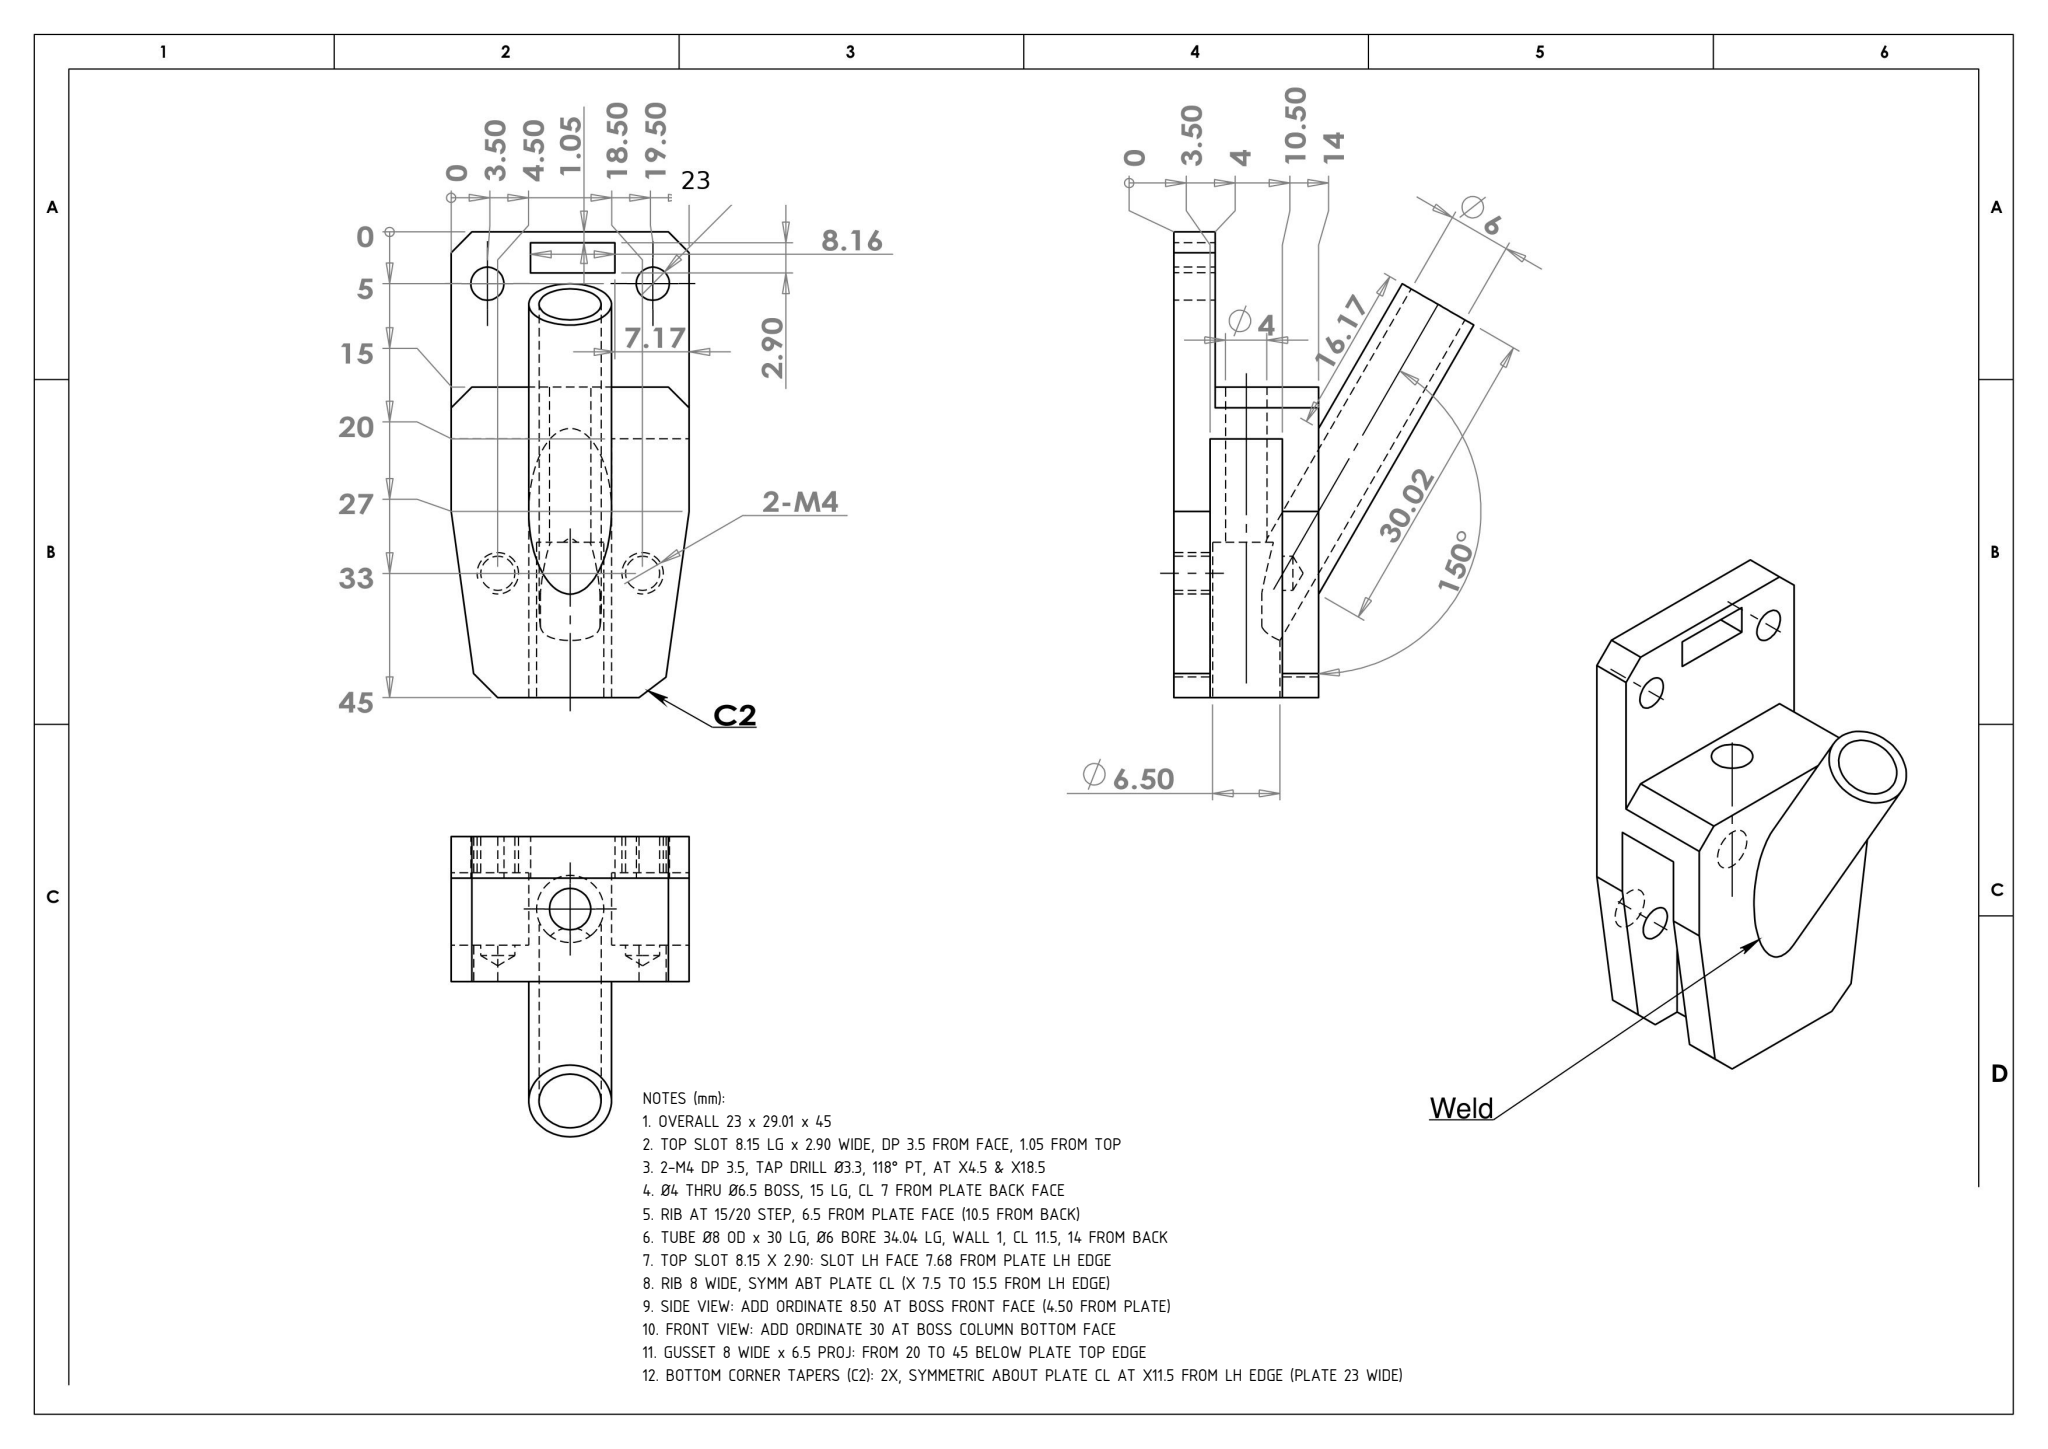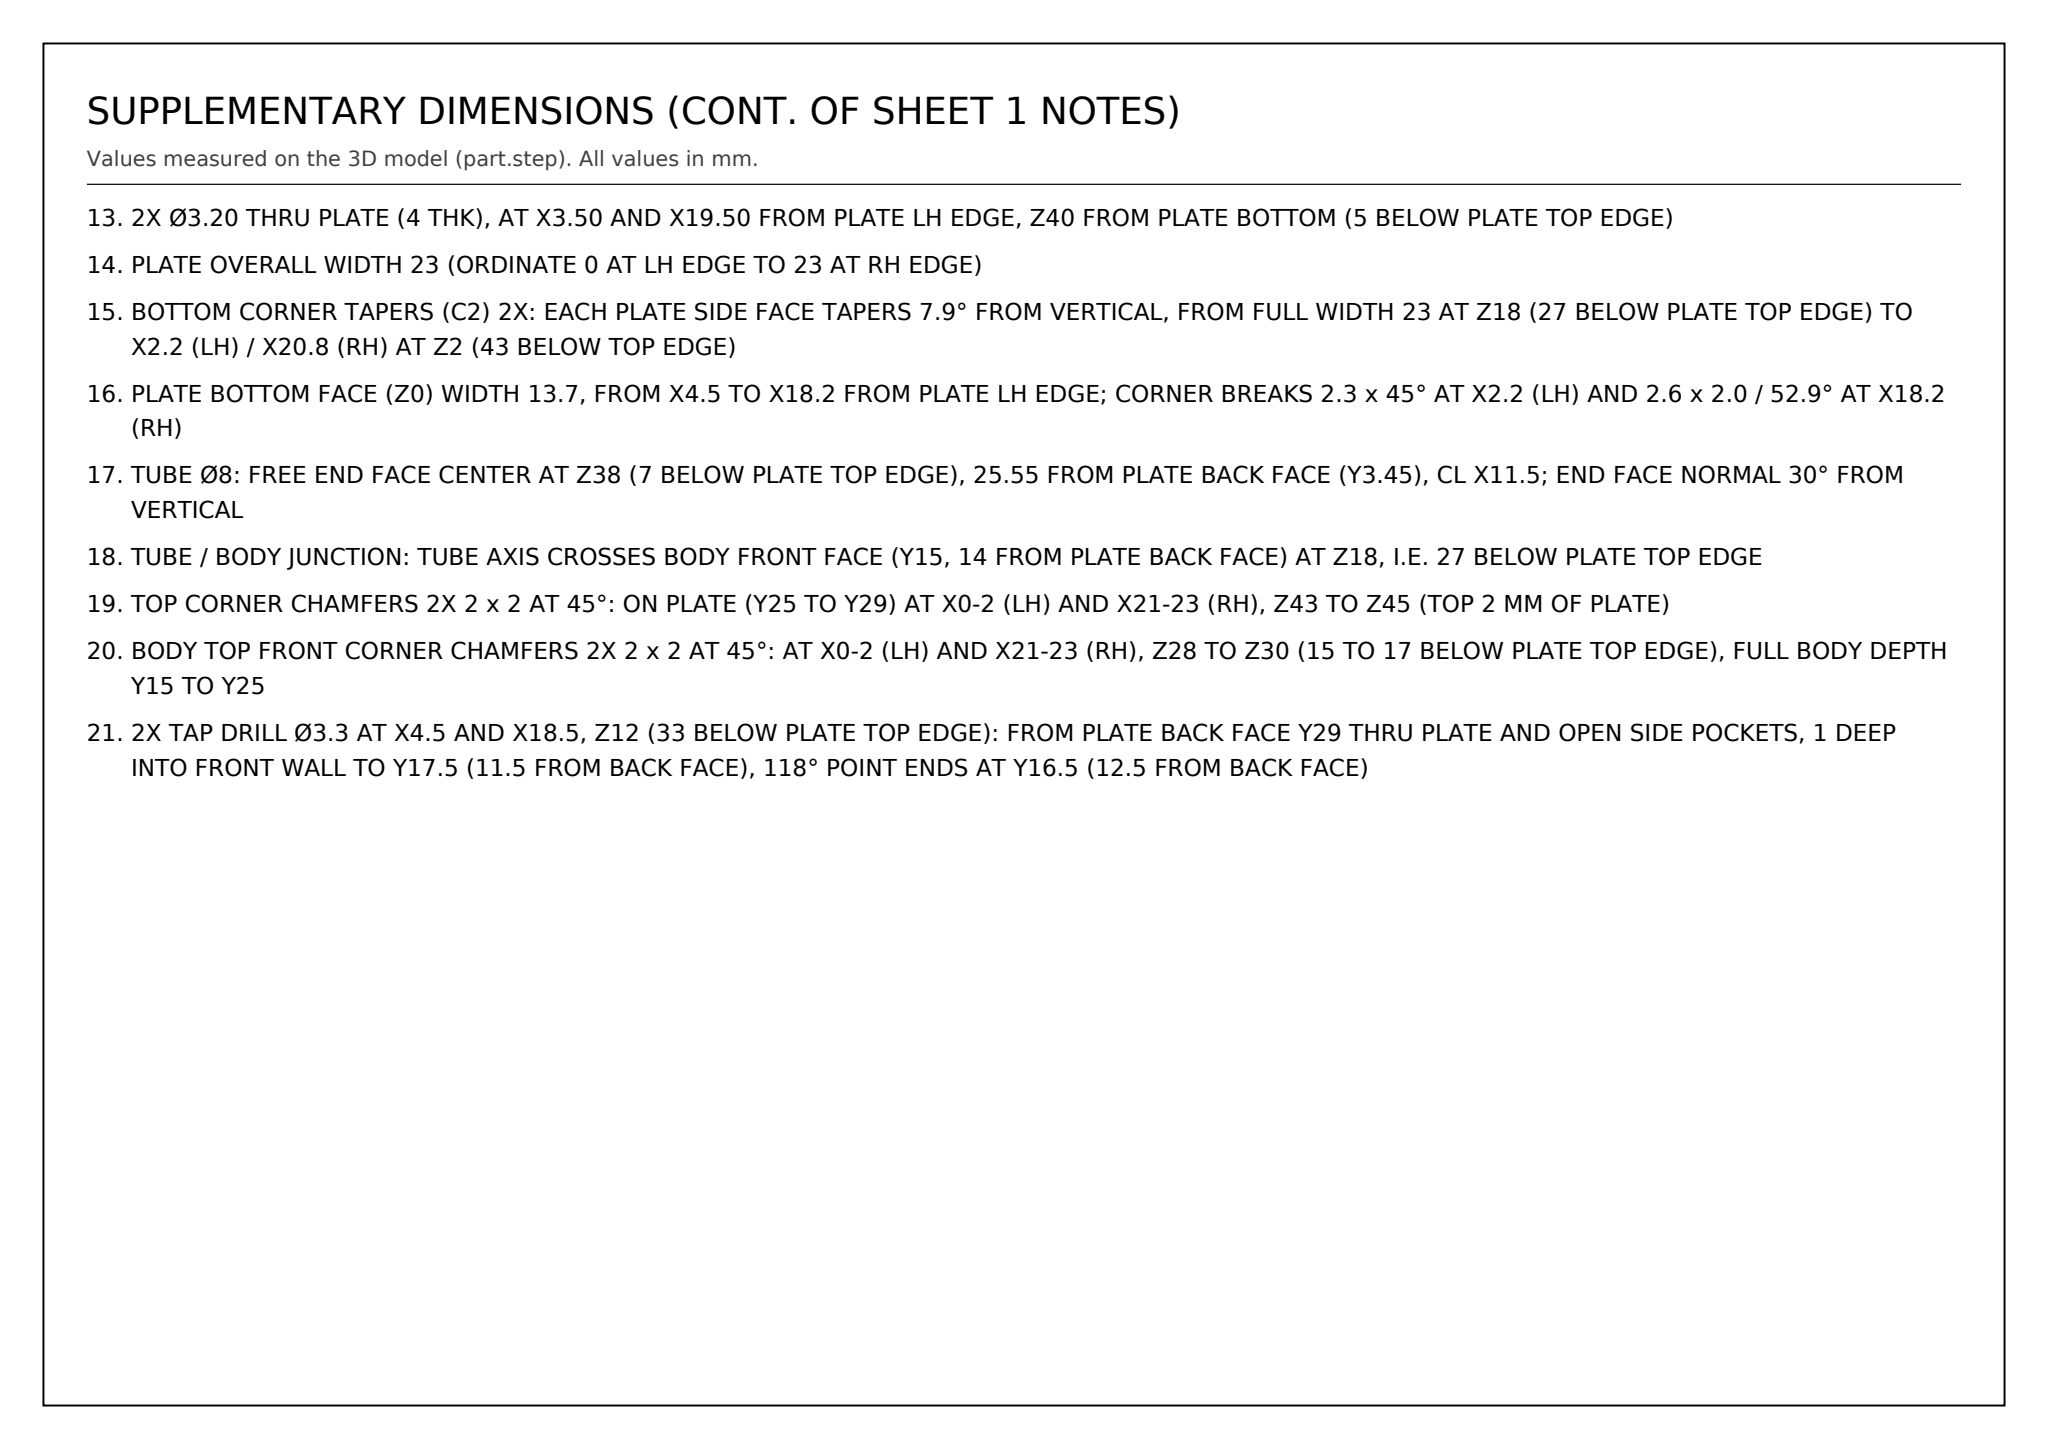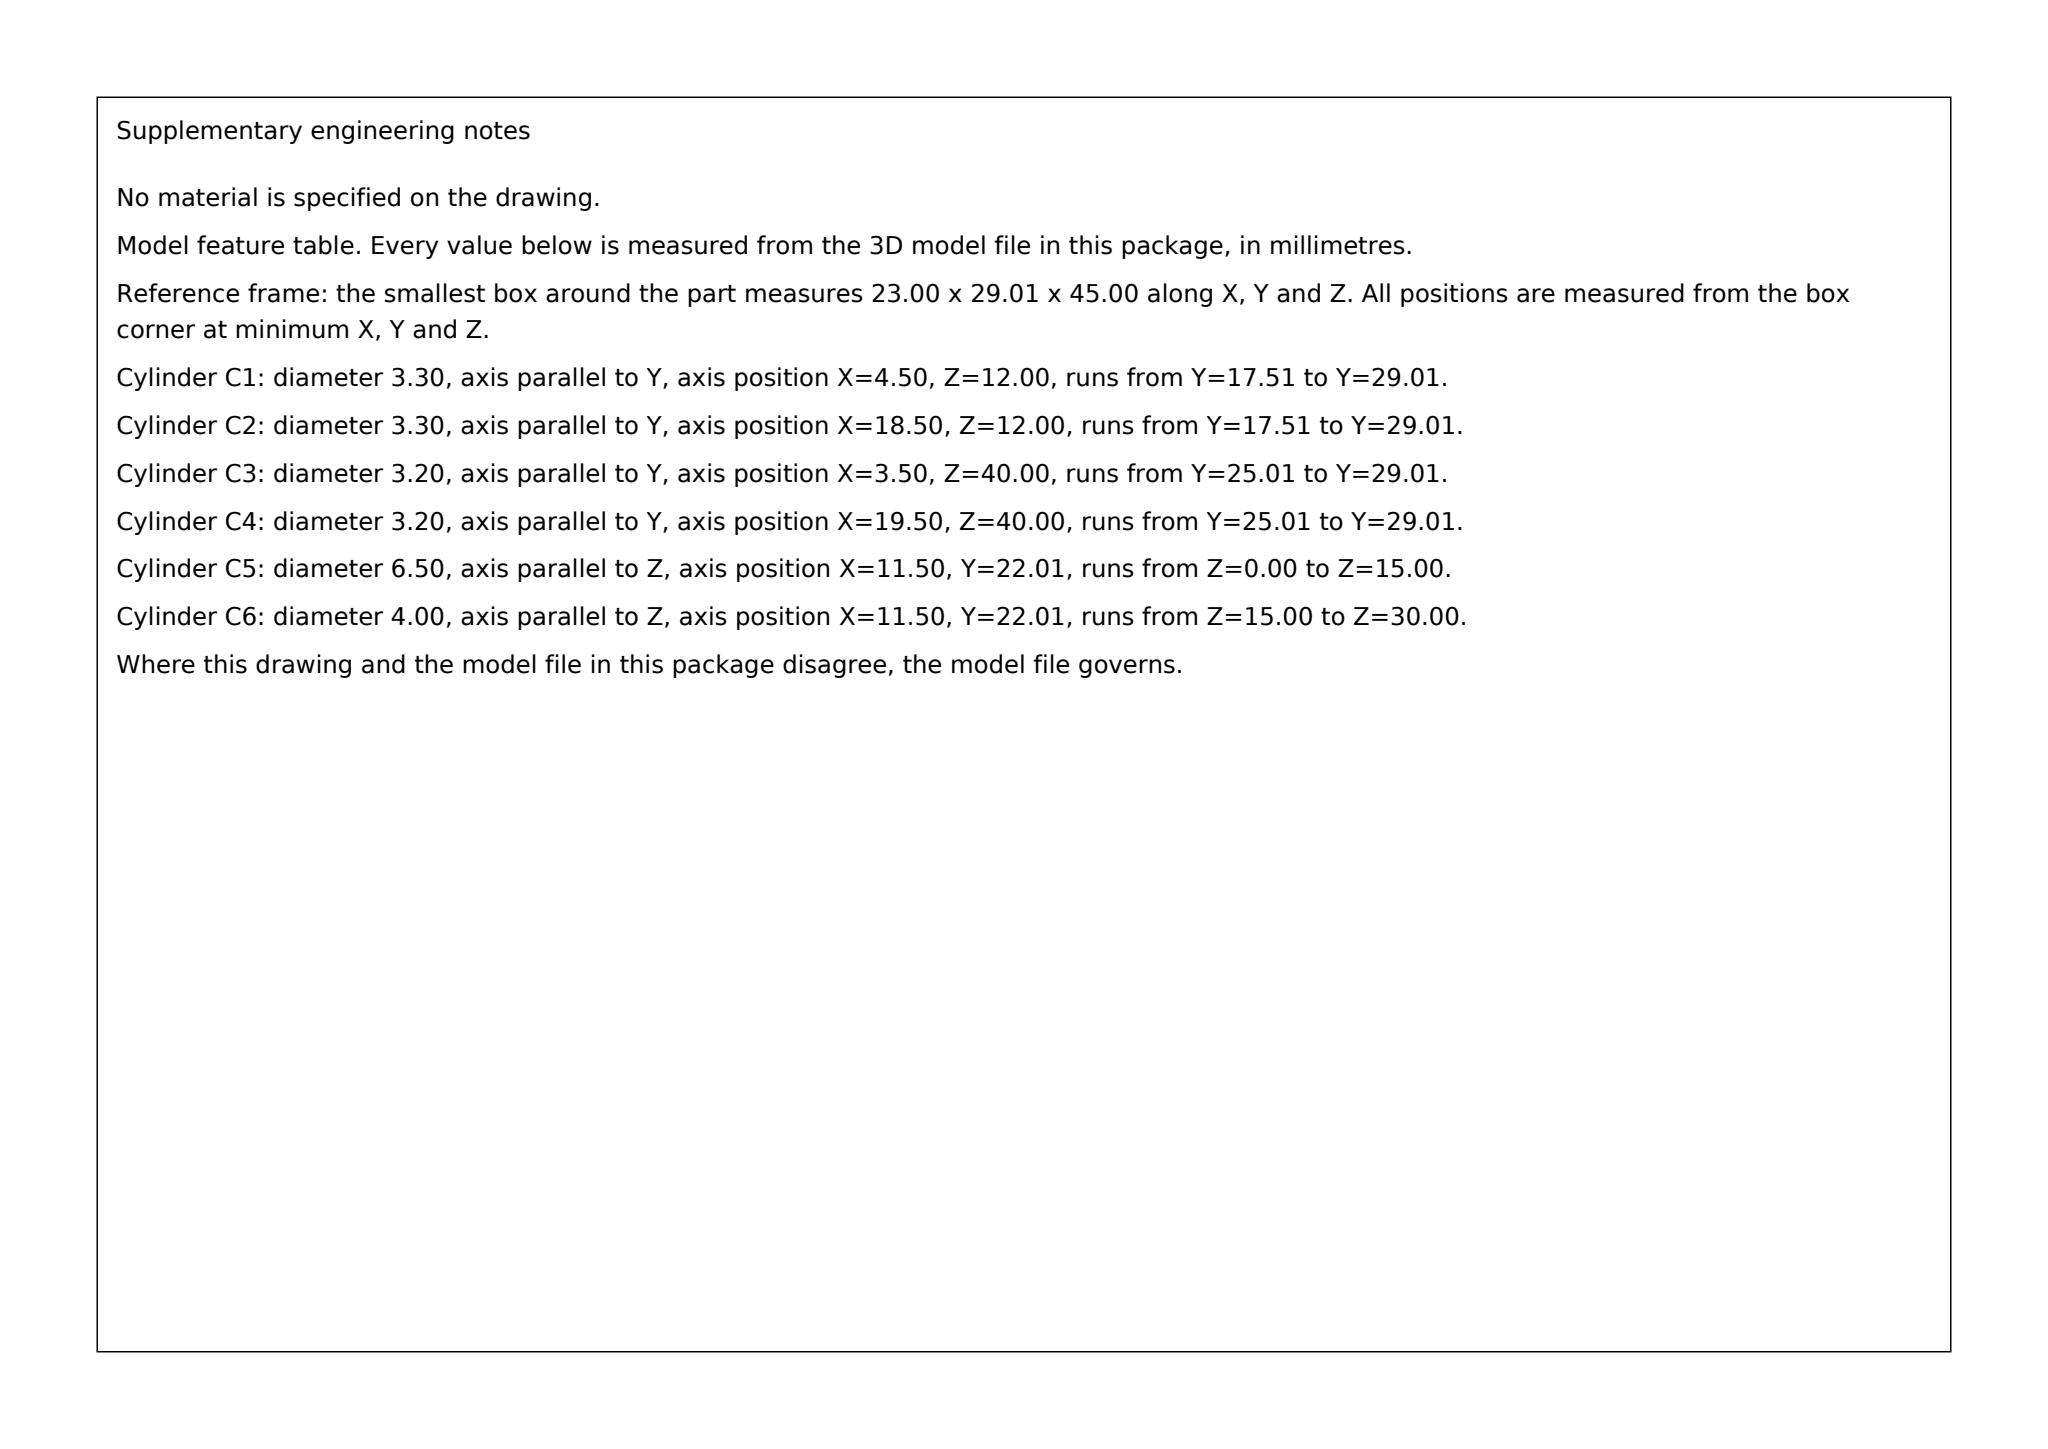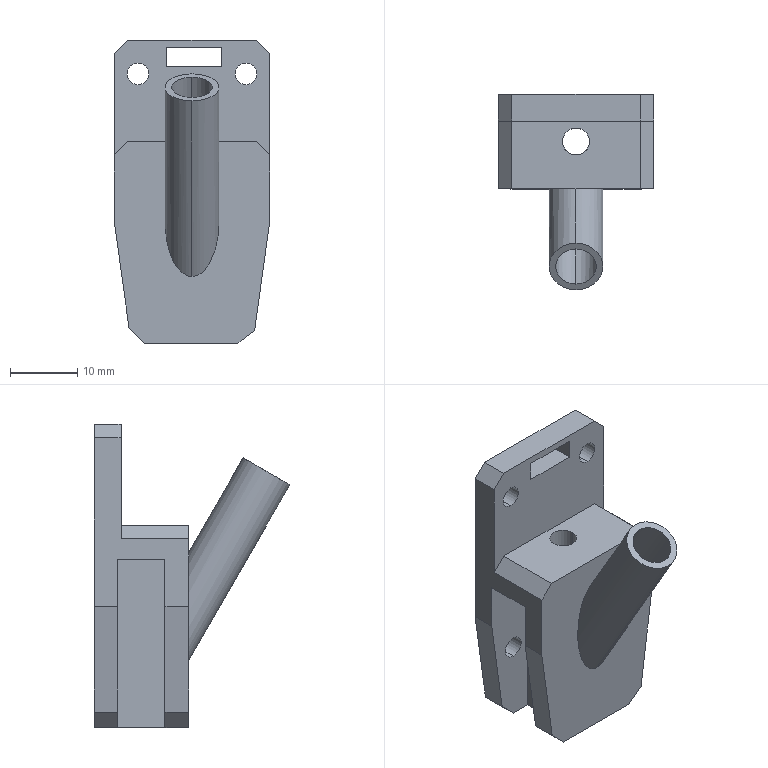Part | SolidWorks | mm | 1 solid | 60 faces | box 23 x 29.01 x 45 mm | volume 7353 mm3 | plane 36 | cylinder 20 | cone 4 | commonest cylinder face diameters 3.3 x8 3.2 x4 4 x2 6.5 x2 8 x2 6 x2
Drawing notes:
OVERALL 23 x 29.01 x 45 | from the solid: bbox_xyz [23.0, 29.011, 45.0]; x faces 0/23, y faces 0/29.01, z faces 0/45
TOP SLOT 8.15 LG x 2.90 WIDE, DP 3.5 FROM FACE, 1.05 FROM TOP | from the solid: x planes 7.68/15.83 = 8.15; z 43.95/41.05 = 2.90, 45-43.95 = 1.05; y 29.01-25.51 = 3.5
2-M4 DP 3.5, TAP DRILL Ø3.3, 118° PT, AT X4.5 & X18.5 | from the solid: Ø3.3 cyls at x=4.5 & 18.5, z=12, L=3.5 (+1.0 lead); cone 118° ref dia 3.3
Ø4 THRU Ø6.5 BOSS, 15 LG, CL 7 FROM PLATE BACK FACE | from the solid: Ø4 and Ø6.5 cyls both at x=11.5, y=22.01, L=15; 29.01-22.01 = 7
RIB AT 15/20 STEP, 6.5 FROM PLATE FACE (10.5 FROM BACK) | from the solid: y planes 18.51 = 10.5 from back 29.01; plate face 25.01 = 4; 10.5-4 = 6.5
TUBE Ø8 OD x 30 LG, Ø6 BORE 34.04 LG, WALL 1, CL 11.5, 14 FROM BACK | from the solid: cyls Ø8 L=30 and Ø6 L=34.04 on same axis [11.5, 15.01]; 29.01-15.01 = 14
TOP SLOT 8.15 X 2.90: SLOT LH FACE 7.68 FROM PLATE LH EDGE | from the solid: x-planes 7.68 & 15.83 (slot faces) vs bbox x=0..23; z 41.05-43.95 = 2.90 high, 1.05 below top z=45
RIB 8 WIDE, SYMM ABT PLATE CL (X 7.5 TO 15.5 FROM LH EDGE) | from the solid: x-planes 7.5 & 15.5 = 8 wide, midpoint 11.5 = bore axis/plate CL (bbox x 0..23)
SIDE VIEW: ADD ORDINATE 8.50 AT BOSS FRONT FACE (4.50 FROM PLATE) | from the solid: y-plane 20.51 with bbox y=29.011 gives 29.011-20.51=8.50 from back datum (ordinate 0); plate front face y=25.01 = 4.0, so boss projects 4.50
FRONT VIEW: ADD ORDINATE 30 AT BOSS COLUMN BOTTOM FACE | from the solid: z-plane 15.0 with bbox z=45 gives 45-15=30 from top datum; Ø8 z-axis cyl at (11.5,15.01) length 30 runs z=15 to 45
GUSSET 8 WIDE x 6.5 PROJ: FROM 20 TO 45 BELOW PLATE TOP EDGE | from the solid: x-planes 7.5 & 15.5 (8 wide, ctr 11.5); y-planes 18.51 & 25.01 (6.5 proj); z-plane 25 (=20 from top face z=45) to z=0 (=45 from top face)
BOTTOM CORNER TAPERS (C2): 2X, SYMMETRIC ABOUT PLATE CL AT X11.5 FROM LH EDGE (PLATE 23 WIDE) | from the solid: bbox_xyz x=23.0 with boss/tube axes at x=11.5 (cylinders dia 6.5/8.0, axis z, pos x=11.5) establishing plate centreline
2X Ø3.20 THRU PLATE (4 THK), AT X3.50 AND X19.50 FROM PLATE LH EDGE, Z40 FROM PLATE BOTTOM (5 BELOW PLATE TOP EDGE) | from the solid: cylinders: [3.2,"y",[3.5,null,40.0],4.0] and [3.2,"y",[19.5,null,40.0],4.0]
PLATE OVERALL WIDTH 23 (ORDINATE 0 AT LH EDGE TO 23 AT RH EDGE) | from the solid: bbox_xyz x = 23.0; axis_planes x = 0.0 and x = 23.0
BOTTOM CORNER TAPERS (C2) 2X: EACH PLATE SIDE FACE TAPERS 7.9° FROM VERTICAL, FROM FULL WIDTH 23 AT Z18 (27 BELOW PLATE TOP EDGE) TO X2.2 (LH) / X20.8 (RH) AT Z2 (43 BELOW TOP EDGE) | from the solid: inclined_planes angle_to_xyz_axes [7.9,90,82.1], bbox_from [0,15,2.3] size [2.2,3.5,15.7] and bbox_from [20.8,15,2.0] size [2.2,3.5,16.0]
PLATE BOTTOM FACE (Z0) WIDTH 13.7, FROM X4.5 TO X18.2 FROM PLATE LH EDGE; CORNER BREAKS 2.3 x 45° AT X2.2 (LH) AND 2.6 x 2.0 / 52.9° AT X18.2 (RH) | from the solid: axis_planes z=0 extent x [4.5,18.2], y [15,29]; inclined_planes [45,90,45] bbox_from [2.2,15,0] size [2.3,3.5,2.3] and [52.9,90,37.1] bbox_from [18.2,15,0] size [2.6,3.5,2.0]
TUBE Ø8: FREE END FACE CENTER AT Z38 (7 BELOW PLATE TOP EDGE), 25.55 FROM PLATE BACK FACE (Y3.45), CL X11.5; END FACE NORMAL 30° FROM VERTICAL | from the solid: inclined_plane angle_to_xyz_axes [90,60,30], bbox_from [7.5,0,36] size [8,6.9,4] (Ø8 tube end face)
TUBE / BODY JUNCTION: TUBE AXIS CROSSES BODY FRONT FACE (Y15, 14 FROM PLATE BACK FACE) AT Z18, I.E. 27 BELOW PLATE TOP EDGE | from the solid: cylinder boss/shaft Ø8 inclined, axis_pos_other_axes [11.5,15.0,null]; axis_planes y=15 extent x [0,23], z [0,30]
TOP CORNER CHAMFERS 2X 2 x 2 AT 45°: ON PLATE (Y25 TO Y29) AT X0-2 (LH) AND X21-23 (RH), Z43 TO Z45 (TOP 2 MM OF PLATE) | from the solid: inclined_planes angle_to_xyz_axes [45,90,45] bbox_from [0,25,43] and [21,25,43], size [2,4,2]
BODY TOP FRONT CORNER CHAMFERS 2X 2 x 2 AT 45°: AT X0-2 (LH) AND X21-23 (RH), Z28 TO Z30 (15 TO 17 BELOW PLATE TOP EDGE), FULL BODY DEPTH Y15 TO Y25 | from the solid: inclined_planes angle_to_xyz_axes [45,90,45] bbox_from [0,15,28] and [21,15,28], size [2,10,2]
2X TAP DRILL Ø3.3 AT X4.5 AND X18.5, Z12 (33 BELOW PLATE TOP EDGE): FROM PLATE BACK FACE Y29 THRU PLATE AND OPEN SIDE POCKETS, 1 DEEP INTO FRONT WALL TO Y17.5 (11.5 FROM BACK FACE), 118° POINT ENDS AT Y16.5 (12.5 FROM BACK FACE) | from the solid: cylinders Ø3.3 y-axis at [4.5,-,12] and [18.5,-,12] from 25.5 to 29.0 and from 17.5 to 18.5; cones 118° ref_dia 3.3 bbox_from y16.5 size [1.7,1.0,3.3]